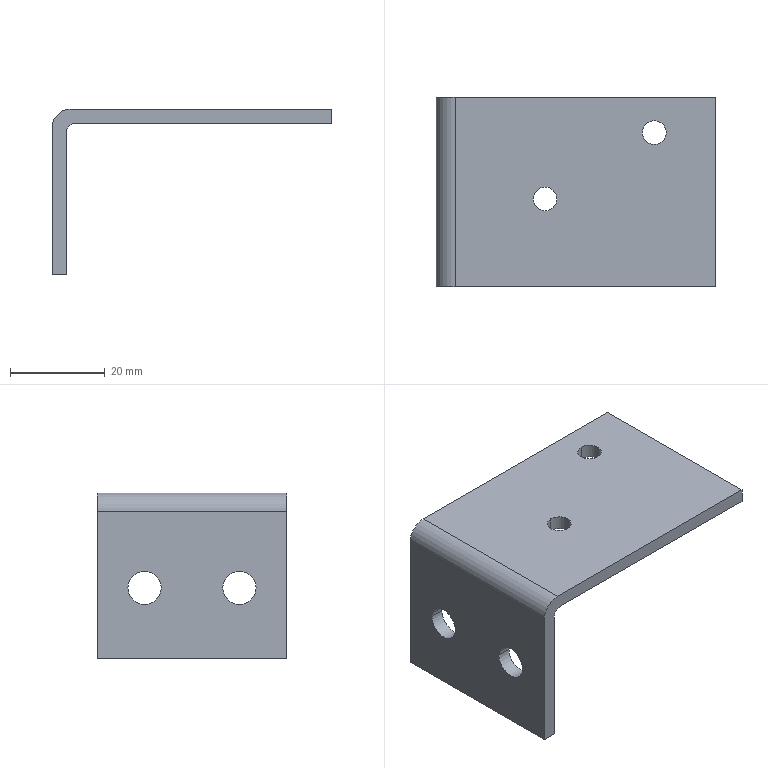Component | SolidWorks | 30-41A-1 | 1 solid | 18 faces | box 59 x 40 x 35 mm | volume 10468 mm3 | cylinder 10 | plane 8 | commonest cylinder face diameters 5 x4 7 x4 8 x1 4 x1
build123d program:
from build123d import *

# Parameters (mm, degrees)
EXTRUDE1_DEPTH        = 20
EXTRUDE1_DEPTH_BACK   = 20
SKETCH2_R             = 3.5
CUT_EXTRUDE1_DEPTH    = 20
M6_TAPPED_HOLE1_D     = 5
M6_TAPPED_HOLE1_DEPTH = 17
M6_TAPPED_HOLE1_TIP   = 1.502


with BuildPart() as part:
    # Sketch1 → Extrude1 (new, two sides: drawn at the far end of the back side and taken through both)
    with BuildSketch(Plane.XY.offset(-EXTRUDE1_DEPTH_BACK)):
        with BuildLine():
            Line((4, 0), (35, 0))
            Line((35, 0), (35, 3))
            Line((35, 3), (5, 3))
            ThreePointArc((5, 3), (3.586, 3.586), (3, 5))
            Line((3, 5), (3, 59))
            Line((3, 59), (0, 59))
            Line((0, 59), (0, 4))
            ThreePointArc((0, 4), (1.172, 1.172), (4, 0))
        make_face()
    extrude(amount=EXTRUDE1_DEPTH + EXTRUDE1_DEPTH_BACK)

    # Sketch2 → Cut-Extrude1 (cut)
    with BuildSketch(Plane(origin=(0, 3, 0), x_dir=(1, 0, 0), z_dir=(0, 1, 0))):
        with Locations(Location((20, 10, 0), (0, 0, 270))):
            Circle(SKETCH2_R)
        with Locations(Location((20, -10, 0), (0, 0, 90))):
            Circle(SKETCH2_R)
    extrude(amount=-CUT_EXTRUDE1_DEPTH, mode=Mode.SUBTRACT)

    # M6 Tapped Hole1
    with Locations(Plane.ZY):
        with Locations((-12.5, 46), (1.5, 23)):
            Hole(M6_TAPPED_HOLE1_D / 2, depth=M6_TAPPED_HOLE1_DEPTH)
            with Locations((0, 0, -(M6_TAPPED_HOLE1_DEPTH + M6_TAPPED_HOLE1_TIP / 2))):  # 118° drill point
                Cone(0, M6_TAPPED_HOLE1_D / 2, M6_TAPPED_HOLE1_TIP, mode=Mode.SUBTRACT)


solid = part.part

# Placed as in the assembly
solid = solid.moved(Location((-429.208, -117.092, 109.188), (90, 0, -90)))
STEP:
#1=CARTESIAN_POINT('',(-15.087,-4.216,4.181));
#2=VERTEX_POINT('',#1);
#3=CARTESIAN_POINT('',(-15.087,-4.019,4.181));
#4=VERTEX_POINT('',#3);
#5=CARTESIAN_POINT('',(-15.087,-4.118,4.181));
#6=DIRECTION('',(-0.,-0.,-1.));
#7=DIRECTION('',(1.,0.,0.));
#8=AXIS2_PLACEMENT_3D('',#5,#6,#7);
#9=CIRCLE('',#8,0.09843);
#10=EDGE_CURVE('',#2,#4,#9,.T.);
#11=ORIENTED_EDGE('',*,*,#10,.T.);
#12=CARTESIAN_POINT('',(-15.087,-4.019,4.299));
#13=VERTEX_POINT('',#12);
#14=CARTESIAN_POINT('',(-15.087,-4.019,4.299));
#15=DIRECTION('',(0.,0.,1.));
#16=VECTOR('',#15,39.37);
#17=LINE('',#14,#16);
#18=EDGE_CURVE('',#4,#13,#17,.T.);
#19=ORIENTED_EDGE('',*,*,#18,.T.);
#20=CARTESIAN_POINT('',(-15.087,-4.216,4.299));
#21=VERTEX_POINT('',#20);
#22=CARTESIAN_POINT('',(-15.087,-4.118,4.299));
#23=DIRECTION('',(0.,0.,1.));
#24=DIRECTION('',(0.,-1.,0.));
#25=AXIS2_PLACEMENT_3D('',#22,#23,#24);
#26=CIRCLE('',#25,0.09843);
#27=EDGE_CURVE('',#13,#21,#26,.T.);
#28=ORIENTED_EDGE('',*,*,#27,.T.);
#29=CARTESIAN_POINT('',(-15.087,-4.216,4.299));
#30=DIRECTION('',(0.,0.,1.));
#31=VECTOR('',#30,39.37);
#32=LINE('',#29,#31);
#33=EDGE_CURVE('',#2,#21,#32,.T.);
#34=ORIENTED_EDGE('',*,*,#33,.F.);
#35=EDGE_LOOP('',(#11,#19,#28,#34));
#36=FACE_OUTER_BOUND('',#35,.T.);
#37=CARTESIAN_POINT('',(-15.087,-4.118,4.299));
#38=DIRECTION('',(0.,0.,1.));
#39=DIRECTION('',(0.,-1.,0.));
#40=AXIS2_PLACEMENT_3D('',#37,#38,#39);
#41=CYLINDRICAL_SURFACE('',#40,0.09843);
#42=ADVANCED_FACE('',(#36),#41,.F.);
#43=CARTESIAN_POINT('',(-15.992,-4.767,4.181));
#44=VERTEX_POINT('',#43);
#45=CARTESIAN_POINT('',(-15.992,-4.571,4.181));
#46=VERTEX_POINT('',#45);
#47=CARTESIAN_POINT('',(-15.992,-4.669,4.181));
#48=DIRECTION('',(-0.,-0.,-1.));
#49=DIRECTION('',(1.,0.,0.));
#50=AXIS2_PLACEMENT_3D('',#47,#48,#49);
#51=CIRCLE('',#50,0.09843);
#52=EDGE_CURVE('',#44,#46,#51,.T.);
#53=ORIENTED_EDGE('',*,*,#52,.T.);
#54=CARTESIAN_POINT('',(-15.992,-4.571,4.299));
#55=VERTEX_POINT('',#54);
#56=CARTESIAN_POINT('',(-15.992,-4.571,4.299));
#57=DIRECTION('',(0.,0.,1.));
#58=VECTOR('',#57,39.37);
#59=LINE('',#56,#58);
#60=EDGE_CURVE('',#46,#55,#59,.T.);
#61=ORIENTED_EDGE('',*,*,#60,.T.);
#62=CARTESIAN_POINT('',(-15.992,-4.767,4.299));
#63=VERTEX_POINT('',#62);
#64=CARTESIAN_POINT('',(-15.992,-4.669,4.299));
#65=DIRECTION('',(0.,0.,1.));
#66=DIRECTION('',(0.,-1.,0.));
#67=AXIS2_PLACEMENT_3D('',#64,#65,#66);
#68=CIRCLE('',#67,0.09843);
#69=EDGE_CURVE('',#55,#63,#68,.T.);
#70=ORIENTED_EDGE('',*,*,#69,.T.);
#71=CARTESIAN_POINT('',(-15.992,-4.767,4.299));
#72=DIRECTION('',(0.,0.,1.));
#73=VECTOR('',#72,39.37);
#74=LINE('',#71,#73);
#75=EDGE_CURVE('',#44,#63,#74,.T.);
#76=ORIENTED_EDGE('',*,*,#75,.F.);
#77=EDGE_LOOP('',(#53,#61,#70,#76));
#78=FACE_OUTER_BOUND('',#77,.T.);
#79=CARTESIAN_POINT('',(-15.992,-4.669,4.299));
#80=DIRECTION('',(0.,0.,1.));
#81=DIRECTION('',(0.,-1.,0.));
#82=AXIS2_PLACEMENT_3D('',#79,#80,#81);
#83=CYLINDRICAL_SURFACE('',#82,0.09843);
#84=ADVANCED_FACE('',(#78),#83,.F.);
#85=CARTESIAN_POINT('',(-16.898,-5.141,3.511));
#86=VERTEX_POINT('',#85);
#87=CARTESIAN_POINT('',(-16.898,-4.866,3.511));
#88=VERTEX_POINT('',#87);
#89=CARTESIAN_POINT('',(-16.898,-5.004,3.511));
#90=DIRECTION('',(-1.,-0.,0.));
#91=DIRECTION('',(0.,1.,0.));
#92=AXIS2_PLACEMENT_3D('',#89,#90,#91);
#93=CIRCLE('',#92,0.1378);
#94=EDGE_CURVE('',#86,#88,#93,.T.);
#95=ORIENTED_EDGE('',*,*,#94,.T.);
#96=CARTESIAN_POINT('',(-16.78,-4.866,3.511));
#97=VERTEX_POINT('',#96);
#98=CARTESIAN_POINT('',(-17.567,-4.866,3.511));
#99=DIRECTION('',(1.,0.,-0.));
#100=VECTOR('',#99,39.37);
#101=LINE('',#98,#100);
#102=EDGE_CURVE('',#88,#97,#101,.T.);
#103=ORIENTED_EDGE('',*,*,#102,.T.);
#104=CARTESIAN_POINT('',(-16.78,-5.141,3.511));
#105=VERTEX_POINT('',#104);
#106=CARTESIAN_POINT('',(-16.78,-5.004,3.511));
#107=DIRECTION('',(1.,0.,-0.));
#108=DIRECTION('',(0.,1.,0.));
#109=AXIS2_PLACEMENT_3D('',#106,#107,#108);
#110=CIRCLE('',#109,0.1378);
#111=EDGE_CURVE('',#97,#105,#110,.T.);
#112=ORIENTED_EDGE('',*,*,#111,.T.);
#113=CARTESIAN_POINT('',(-17.567,-5.141,3.511));
#114=DIRECTION('',(1.,0.,-0.));
#115=VECTOR('',#114,39.37);
#116=LINE('',#113,#115);
#117=EDGE_CURVE('',#86,#105,#116,.T.);
#118=ORIENTED_EDGE('',*,*,#117,.F.);
#119=EDGE_LOOP('',(#95,#103,#112,#118));
#120=FACE_OUTER_BOUND('',#119,.T.);
#121=CARTESIAN_POINT('',(-17.567,-5.004,3.511));
#122=DIRECTION('',(1.,0.,-0.));
#123=DIRECTION('',(0.,-1.,0.));
#124=AXIS2_PLACEMENT_3D('',#121,#122,#123);
#125=CYLINDRICAL_SURFACE('',#124,0.1378);
#126=ADVANCED_FACE('',(#120),#125,.F.);
#127=CARTESIAN_POINT('',(-16.898,-4.354,3.511));
#128=VERTEX_POINT('',#127);
#129=CARTESIAN_POINT('',(-16.898,-4.078,3.511));
#130=VERTEX_POINT('',#129);
#131=CARTESIAN_POINT('',(-16.898,-4.216,3.511));
#132=DIRECTION('',(-1.,-0.,0.));
#133=DIRECTION('',(0.,1.,0.));
#134=AXIS2_PLACEMENT_3D('',#131,#132,#133);
#135=CIRCLE('',#134,0.1378);
#136=EDGE_CURVE('',#128,#130,#135,.T.);
#137=ORIENTED_EDGE('',*,*,#136,.T.);
#138=CARTESIAN_POINT('',(-16.78,-4.078,3.511));
#139=VERTEX_POINT('',#138);
#140=CARTESIAN_POINT('',(-17.567,-4.078,3.511));
#141=DIRECTION('',(1.,0.,-0.));
#142=VECTOR('',#141,39.37);
#143=LINE('',#140,#142);
#144=EDGE_CURVE('',#130,#139,#143,.T.);
#145=ORIENTED_EDGE('',*,*,#144,.T.);
#146=CARTESIAN_POINT('',(-16.78,-4.354,3.511));
#147=VERTEX_POINT('',#146);
#148=CARTESIAN_POINT('',(-16.78,-4.216,3.511));
#149=DIRECTION('',(1.,0.,-0.));
#150=DIRECTION('',(0.,-1.,0.));
#151=AXIS2_PLACEMENT_3D('',#148,#149,#150);
#152=CIRCLE('',#151,0.1378);
#153=EDGE_CURVE('',#139,#147,#152,.T.);
#154=ORIENTED_EDGE('',*,*,#153,.T.);
#155=CARTESIAN_POINT('',(-17.567,-4.354,3.511));
#156=DIRECTION('',(1.,0.,-0.));
#157=VECTOR('',#156,39.37);
#158=LINE('',#155,#157);
#159=EDGE_CURVE('',#128,#147,#158,.T.);
#160=ORIENTED_EDGE('',*,*,#159,.F.);
#161=EDGE_LOOP('',(#137,#145,#154,#160));
#162=FACE_OUTER_BOUND('',#161,.T.);
#163=CARTESIAN_POINT('',(-17.567,-4.216,3.511));
#164=DIRECTION('',(1.,0.,-0.));
#165=DIRECTION('',(0.,-1.,0.));
#166=AXIS2_PLACEMENT_3D('',#163,#164,#165);
#167=CYLINDRICAL_SURFACE('',#166,0.1378);
#168=ADVANCED_FACE('',(#162),#167,.F.);
#169=CARTESIAN_POINT('',(-16.78,-3.823,2.921));
#170=VERTEX_POINT('',#169);
#171=CARTESIAN_POINT('',(-16.78,-5.397,2.921));
#172=VERTEX_POINT('',#171);
#173=CARTESIAN_POINT('',(-16.78,-3.823,2.921));
#174=DIRECTION('',(0.,-1.,0.));
#175=VECTOR('',#174,39.37);
#176=LINE('',#173,#175);
#177=EDGE_CURVE('',#170,#172,#176,.T.);
#178=ORIENTED_EDGE('',*,*,#177,.T.);
#179=CARTESIAN_POINT('',(-16.898,-5.397,2.921));
#180=VERTEX_POINT('',#179);
#181=CARTESIAN_POINT('',(-16.898,-5.397,2.921));
#182=DIRECTION('',(1.,0.,-0.));
#183=VECTOR('',#182,39.37);
#184=LINE('',#181,#183);
#185=EDGE_CURVE('',#180,#172,#184,.T.);
#186=ORIENTED_EDGE('',*,*,#185,.F.);
#187=CARTESIAN_POINT('',(-16.898,-3.823,2.921));
#188=VERTEX_POINT('',#187);
#189=CARTESIAN_POINT('',(-16.898,-3.823,2.921));
#190=DIRECTION('',(0.,-1.,0.));
#191=VECTOR('',#190,39.37);
#192=LINE('',#189,#191);
#193=EDGE_CURVE('',#188,#180,#192,.T.);
#194=ORIENTED_EDGE('',*,*,#193,.F.);
#195=CARTESIAN_POINT('',(-16.898,-3.823,2.921));
#196=DIRECTION('',(1.,0.,-0.));
#197=VECTOR('',#196,39.37);
#198=LINE('',#195,#197);
#199=EDGE_CURVE('',#188,#170,#198,.T.);
#200=ORIENTED_EDGE('',*,*,#199,.T.);
#201=EDGE_LOOP('',(#178,#186,#194,#200));
#202=FACE_OUTER_BOUND('',#201,.T.);
#203=CARTESIAN_POINT('',(-16.898,-3.823,2.921));
#204=DIRECTION('',(-0.,-0.,-1.));
#205=DIRECTION('',(-0.,1.,-0.));
#206=AXIS2_PLACEMENT_3D('',#203,#204,#205);
#207=PLANE('',#206);
#208=ADVANCED_FACE('',(#202),#207,.T.);
#209=ORIENTED_EDGE('',*,*,#94,.F.);
#210=CARTESIAN_POINT('',(-16.898,-5.004,3.511));
#211=DIRECTION('',(-1.,-0.,0.));
#212=DIRECTION('',(0.,1.,0.));
#213=AXIS2_PLACEMENT_3D('',#210,#211,#212);
#214=CIRCLE('',#213,0.1378);
#215=EDGE_CURVE('',#88,#86,#214,.T.);
#216=ORIENTED_EDGE('',*,*,#215,.F.);
#217=EDGE_LOOP('',(#209,#216));
#218=FACE_BOUND('',#217,.T.);
#219=ORIENTED_EDGE('',*,*,#136,.F.);
#220=CARTESIAN_POINT('',(-16.898,-4.216,3.511));
#221=DIRECTION('',(-1.,-0.,0.));
#222=DIRECTION('',(0.,1.,0.));
#223=AXIS2_PLACEMENT_3D('',#220,#221,#222);
#224=CIRCLE('',#223,0.1378);
#225=EDGE_CURVE('',#130,#128,#224,.T.);
#226=ORIENTED_EDGE('',*,*,#225,.F.);
#227=EDGE_LOOP('',(#219,#226));
#228=FACE_BOUND('',#227,.T.);
#229=ORIENTED_EDGE('',*,*,#193,.T.);
#230=CARTESIAN_POINT('',(-16.898,-5.397,4.141));
#231=VERTEX_POINT('',#230);
#232=CARTESIAN_POINT('',(-16.898,-5.397,4.141));
#233=DIRECTION('',(-0.,-0.,-1.));
#234=VECTOR('',#233,39.37);
#235=LINE('',#232,#234);
#236=EDGE_CURVE('',#231,#180,#235,.T.);
#237=ORIENTED_EDGE('',*,*,#236,.F.);
#238=CARTESIAN_POINT('',(-16.898,-3.823,4.141));
#239=VERTEX_POINT('',#238);
#240=CARTESIAN_POINT('',(-16.898,-3.823,4.141));
#241=DIRECTION('',(0.,-1.,0.));
#242=VECTOR('',#241,39.37);
#243=LINE('',#240,#242);
#244=EDGE_CURVE('',#239,#231,#243,.T.);
#245=ORIENTED_EDGE('',*,*,#244,.F.);
#246=CARTESIAN_POINT('',(-16.898,-3.823,4.141));
#247=DIRECTION('',(-0.,-0.,-1.));
#248=VECTOR('',#247,39.37);
#249=LINE('',#246,#248);
#250=EDGE_CURVE('',#239,#188,#249,.T.);
#251=ORIENTED_EDGE('',*,*,#250,.T.);
#252=EDGE_LOOP('',(#229,#237,#245,#251));
#253=FACE_OUTER_BOUND('',#252,.T.);
#254=CARTESIAN_POINT('',(-16.898,-3.823,4.141));
#255=DIRECTION('',(-1.,-0.,0.));
#256=DIRECTION('',(-0.,1.,-0.));
#257=AXIS2_PLACEMENT_3D('',#254,#255,#256);
#258=PLANE('',#257);
#259=ADVANCED_FACE('',(#218,#228,#253),#258,.T.);
#260=ORIENTED_EDGE('',*,*,#244,.T.);
#261=CARTESIAN_POINT('',(-16.74,-5.397,4.299));
#262=VERTEX_POINT('',#261);
#263=CARTESIAN_POINT('',(-16.74,-5.397,4.141));
#264=DIRECTION('',(0.,-1.,0.));
#265=DIRECTION('',(0.,0.,1.));
#266=AXIS2_PLACEMENT_3D('',#263,#264,#265);
#267=CIRCLE('',#266,0.1575);
#268=EDGE_CURVE('',#262,#231,#267,.T.);
#269=ORIENTED_EDGE('',*,*,#268,.F.);
#270=CARTESIAN_POINT('',(-16.74,-3.823,4.299));
#271=VERTEX_POINT('',#270);
#272=CARTESIAN_POINT('',(-16.74,-3.823,4.299));
#273=DIRECTION('',(0.,-1.,0.));
#274=VECTOR('',#273,39.37);
#275=LINE('',#272,#274);
#276=EDGE_CURVE('',#271,#262,#275,.T.);
#277=ORIENTED_EDGE('',*,*,#276,.F.);
#278=CARTESIAN_POINT('',(-16.74,-3.823,4.141));
#279=DIRECTION('',(0.,-1.,0.));
#280=DIRECTION('',(0.,0.,1.));
#281=AXIS2_PLACEMENT_3D('',#278,#279,#280);
#282=CIRCLE('',#281,0.1575);
#283=EDGE_CURVE('',#271,#239,#282,.T.);
#284=ORIENTED_EDGE('',*,*,#283,.T.);
#285=EDGE_LOOP('',(#260,#269,#277,#284));
#286=FACE_OUTER_BOUND('',#285,.T.);
#287=CARTESIAN_POINT('',(-16.74,-3.823,4.141));
#288=DIRECTION('',(0.,-1.,0.));
#289=DIRECTION('',(0.,0.,-1.));
#290=AXIS2_PLACEMENT_3D('',#287,#288,#289);
#291=CYLINDRICAL_SURFACE('',#290,0.1575);
#292=ADVANCED_FACE('',(#286),#291,.T.);
#293=CARTESIAN_POINT('',(-15.087,-4.118,4.299));
#294=DIRECTION('',(0.,0.,1.));
#295=DIRECTION('',(0.,-1.,0.));
#296=AXIS2_PLACEMENT_3D('',#293,#294,#295);
#297=CIRCLE('',#296,0.09843);
#298=EDGE_CURVE('',#21,#13,#297,.T.);
#299=ORIENTED_EDGE('',*,*,#298,.F.);
#300=ORIENTED_EDGE('',*,*,#27,.F.);
#301=EDGE_LOOP('',(#299,#300));
#302=FACE_BOUND('',#301,.T.);
#303=CARTESIAN_POINT('',(-15.992,-4.669,4.299));
#304=DIRECTION('',(0.,0.,1.));
#305=DIRECTION('',(0.,-1.,0.));
#306=AXIS2_PLACEMENT_3D('',#303,#304,#305);
#307=CIRCLE('',#306,0.09843);
#308=EDGE_CURVE('',#63,#55,#307,.T.);
#309=ORIENTED_EDGE('',*,*,#308,.F.);
#310=ORIENTED_EDGE('',*,*,#69,.F.);
#311=EDGE_LOOP('',(#309,#310));
#312=FACE_BOUND('',#311,.T.);
#313=ORIENTED_EDGE('',*,*,#276,.T.);
#314=CARTESIAN_POINT('',(-14.575,-5.397,4.299));
#315=VERTEX_POINT('',#314);
#316=CARTESIAN_POINT('',(-16.74,-5.397,4.299));
#317=DIRECTION('',(-1.,-0.,0.));
#318=VECTOR('',#317,39.37);
#319=LINE('',#316,#318);
#320=EDGE_CURVE('',#315,#262,#319,.T.);
#321=ORIENTED_EDGE('',*,*,#320,.F.);
#322=CARTESIAN_POINT('',(-14.575,-3.823,4.299));
#323=VERTEX_POINT('',#322);
#324=CARTESIAN_POINT('',(-14.575,-3.823,4.299));
#325=DIRECTION('',(0.,-1.,0.));
#326=VECTOR('',#325,39.37);
#327=LINE('',#324,#326);
#328=EDGE_CURVE('',#323,#315,#327,.T.);
#329=ORIENTED_EDGE('',*,*,#328,.F.);
#330=CARTESIAN_POINT('',(-16.74,-3.823,4.299));
#331=DIRECTION('',(-1.,-0.,0.));
#332=VECTOR('',#331,39.37);
#333=LINE('',#330,#332);
#334=EDGE_CURVE('',#323,#271,#333,.T.);
#335=ORIENTED_EDGE('',*,*,#334,.T.);
#336=EDGE_LOOP('',(#313,#321,#329,#335));
#337=FACE_OUTER_BOUND('',#336,.T.);
#338=CARTESIAN_POINT('',(-16.74,-3.823,4.299));
#339=DIRECTION('',(0.,0.,1.));
#340=DIRECTION('',(0.,-1.,0.));
#341=AXIS2_PLACEMENT_3D('',#338,#339,#340);
#342=PLANE('',#341);
#343=ADVANCED_FACE('',(#302,#312,#337),#342,.T.);
#344=ORIENTED_EDGE('',*,*,#328,.T.);
#345=CARTESIAN_POINT('',(-14.575,-5.397,4.181));
#346=VERTEX_POINT('',#345);
#347=CARTESIAN_POINT('',(-14.575,-5.397,4.299));
#348=DIRECTION('',(0.,0.,1.));
#349=VECTOR('',#348,39.37);
#350=LINE('',#347,#349);
#351=EDGE_CURVE('',#346,#315,#350,.T.);
#352=ORIENTED_EDGE('',*,*,#351,.F.);
#353=CARTESIAN_POINT('',(-14.575,-3.823,4.181));
#354=VERTEX_POINT('',#353);
#355=CARTESIAN_POINT('',(-14.575,-3.823,4.181));
#356=DIRECTION('',(0.,-1.,0.));
#357=VECTOR('',#356,39.37);
#358=LINE('',#355,#357);
#359=EDGE_CURVE('',#354,#346,#358,.T.);
#360=ORIENTED_EDGE('',*,*,#359,.F.);
#361=CARTESIAN_POINT('',(-14.575,-3.823,4.299));
#362=DIRECTION('',(0.,0.,1.));
#363=VECTOR('',#362,39.37);
#364=LINE('',#361,#363);
#365=EDGE_CURVE('',#354,#323,#364,.T.);
#366=ORIENTED_EDGE('',*,*,#365,.T.);
#367=EDGE_LOOP('',(#344,#352,#360,#366));
#368=FACE_OUTER_BOUND('',#367,.T.);
#369=CARTESIAN_POINT('',(-14.575,-3.823,4.299));
#370=DIRECTION('',(1.,0.,-0.));
#371=DIRECTION('',(0.,-1.,0.));
#372=AXIS2_PLACEMENT_3D('',#369,#370,#371);
#373=PLANE('',#372);
#374=ADVANCED_FACE('',(#368),#373,.T.);
#375=ORIENTED_EDGE('',*,*,#10,.F.);
#376=CARTESIAN_POINT('',(-15.087,-4.118,4.181));
#377=DIRECTION('',(-0.,-0.,-1.));
#378=DIRECTION('',(1.,0.,0.));
#379=AXIS2_PLACEMENT_3D('',#376,#377,#378);
#380=CIRCLE('',#379,0.09843);
#381=EDGE_CURVE('',#4,#2,#380,.T.);
#382=ORIENTED_EDGE('',*,*,#381,.F.);
#383=EDGE_LOOP('',(#375,#382));
#384=FACE_BOUND('',#383,.T.);
#385=ORIENTED_EDGE('',*,*,#52,.F.);
#386=CARTESIAN_POINT('',(-15.992,-4.669,4.181));
#387=DIRECTION('',(-0.,-0.,-1.));
#388=DIRECTION('',(1.,0.,0.));
#389=AXIS2_PLACEMENT_3D('',#386,#387,#388);
#390=CIRCLE('',#389,0.09843);
#391=EDGE_CURVE('',#46,#44,#390,.T.);
#392=ORIENTED_EDGE('',*,*,#391,.F.);
#393=EDGE_LOOP('',(#385,#392));
#394=FACE_BOUND('',#393,.T.);
#395=ORIENTED_EDGE('',*,*,#359,.T.);
#396=CARTESIAN_POINT('',(-16.701,-5.397,4.181));
#397=VERTEX_POINT('',#396);
#398=CARTESIAN_POINT('',(-14.575,-5.397,4.181));
#399=DIRECTION('',(1.,0.,-0.));
#400=VECTOR('',#399,39.37);
#401=LINE('',#398,#400);
#402=EDGE_CURVE('',#397,#346,#401,.T.);
#403=ORIENTED_EDGE('',*,*,#402,.F.);
#404=CARTESIAN_POINT('',(-16.701,-3.823,4.181));
#405=VERTEX_POINT('',#404);
#406=CARTESIAN_POINT('',(-16.701,-3.823,4.181));
#407=DIRECTION('',(0.,-1.,0.));
#408=VECTOR('',#407,39.37);
#409=LINE('',#406,#408);
#410=EDGE_CURVE('',#405,#397,#409,.T.);
#411=ORIENTED_EDGE('',*,*,#410,.F.);
#412=CARTESIAN_POINT('',(-14.575,-3.823,4.181));
#413=DIRECTION('',(1.,0.,-0.));
#414=VECTOR('',#413,39.37);
#415=LINE('',#412,#414);
#416=EDGE_CURVE('',#405,#354,#415,.T.);
#417=ORIENTED_EDGE('',*,*,#416,.T.);
#418=EDGE_LOOP('',(#395,#403,#411,#417));
#419=FACE_OUTER_BOUND('',#418,.T.);
#420=CARTESIAN_POINT('',(-14.575,-3.823,4.181));
#421=DIRECTION('',(-0.,-0.,-1.));
#422=DIRECTION('',(1.,0.,-0.));
#423=AXIS2_PLACEMENT_3D('',#420,#421,#422);
#424=PLANE('',#423);
#425=ADVANCED_FACE('',(#384,#394,#419),#424,.T.);
#426=ORIENTED_EDGE('',*,*,#410,.T.);
#427=CARTESIAN_POINT('',(-16.78,-5.397,4.102));
#428=VERTEX_POINT('',#427);
#429=CARTESIAN_POINT('',(-16.701,-5.397,4.102));
#430=DIRECTION('',(-0.,1.,-0.));
#431=DIRECTION('',(0.,0.,1.));
#432=AXIS2_PLACEMENT_3D('',#429,#430,#431);
#433=CIRCLE('',#432,0.07874);
#434=EDGE_CURVE('',#428,#397,#433,.T.);
#435=ORIENTED_EDGE('',*,*,#434,.F.);
#436=CARTESIAN_POINT('',(-16.78,-3.823,4.102));
#437=VERTEX_POINT('',#436);
#438=CARTESIAN_POINT('',(-16.78,-3.823,4.102));
#439=DIRECTION('',(0.,-1.,0.));
#440=VECTOR('',#439,39.37);
#441=LINE('',#438,#440);
#442=EDGE_CURVE('',#437,#428,#441,.T.);
#443=ORIENTED_EDGE('',*,*,#442,.F.);
#444=CARTESIAN_POINT('',(-16.701,-3.823,4.102));
#445=DIRECTION('',(-0.,1.,-0.));
#446=DIRECTION('',(0.,0.,1.));
#447=AXIS2_PLACEMENT_3D('',#444,#445,#446);
#448=CIRCLE('',#447,0.07874);
#449=EDGE_CURVE('',#437,#405,#448,.T.);
#450=ORIENTED_EDGE('',*,*,#449,.T.);
#451=EDGE_LOOP('',(#426,#435,#443,#450));
#452=FACE_OUTER_BOUND('',#451,.T.);
#453=CARTESIAN_POINT('',(-16.701,-3.823,4.102));
#454=DIRECTION('',(0.,-1.,0.));
#455=DIRECTION('',(0.,0.,-1.));
#456=AXIS2_PLACEMENT_3D('',#453,#454,#455);
#457=CYLINDRICAL_SURFACE('',#456,0.07874);
#458=ADVANCED_FACE('',(#452),#457,.F.);
#459=CARTESIAN_POINT('',(-16.78,-5.004,3.511));
#460=DIRECTION('',(1.,0.,-0.));
#461=DIRECTION('',(0.,1.,0.));
#462=AXIS2_PLACEMENT_3D('',#459,#460,#461);
#463=CIRCLE('',#462,0.1378);
#464=EDGE_CURVE('',#105,#97,#463,.T.);
#465=ORIENTED_EDGE('',*,*,#464,.F.);
#466=ORIENTED_EDGE('',*,*,#111,.F.);
#467=EDGE_LOOP('',(#465,#466));
#468=FACE_BOUND('',#467,.T.);
#469=CARTESIAN_POINT('',(-16.78,-4.216,3.511));
#470=DIRECTION('',(1.,0.,-0.));
#471=DIRECTION('',(0.,-1.,0.));
#472=AXIS2_PLACEMENT_3D('',#469,#470,#471);
#473=CIRCLE('',#472,0.1378);
#474=EDGE_CURVE('',#147,#139,#473,.T.);
#475=ORIENTED_EDGE('',*,*,#474,.F.);
#476=ORIENTED_EDGE('',*,*,#153,.F.);
#477=EDGE_LOOP('',(#475,#476));
#478=FACE_BOUND('',#477,.T.);
#479=ORIENTED_EDGE('',*,*,#442,.T.);
#480=CARTESIAN_POINT('',(-16.78,-5.397,4.102));
#481=DIRECTION('',(0.,0.,1.));
#482=VECTOR('',#481,39.37);
#483=LINE('',#480,#482);
#484=EDGE_CURVE('',#172,#428,#483,.T.);
#485=ORIENTED_EDGE('',*,*,#484,.F.);
#486=ORIENTED_EDGE('',*,*,#177,.F.);
#487=CARTESIAN_POINT('',(-16.78,-3.823,4.102));
#488=DIRECTION('',(0.,0.,1.));
#489=VECTOR('',#488,39.37);
#490=LINE('',#487,#489);
#491=EDGE_CURVE('',#170,#437,#490,.T.);
#492=ORIENTED_EDGE('',*,*,#491,.T.);
#493=EDGE_LOOP('',(#479,#485,#486,#492));
#494=FACE_OUTER_BOUND('',#493,.T.);
#495=CARTESIAN_POINT('',(-16.78,-3.823,4.102));
#496=DIRECTION('',(1.,0.,-0.));
#497=DIRECTION('',(0.,-1.,0.));
#498=AXIS2_PLACEMENT_3D('',#495,#496,#497);
#499=PLANE('',#498);
#500=ADVANCED_FACE('',(#468,#478,#494),#499,.T.);
#501=ORIENTED_EDGE('',*,*,#199,.F.);
#502=ORIENTED_EDGE('',*,*,#250,.F.);
#503=ORIENTED_EDGE('',*,*,#283,.F.);
#504=ORIENTED_EDGE('',*,*,#334,.F.);
#505=ORIENTED_EDGE('',*,*,#365,.F.);
#506=ORIENTED_EDGE('',*,*,#416,.F.);
#507=ORIENTED_EDGE('',*,*,#449,.F.);
#508=ORIENTED_EDGE('',*,*,#491,.F.);
#509=EDGE_LOOP('',(#501,#502,#503,#504,#505,#506,#507,#508));
#510=FACE_OUTER_BOUND('',#509,.T.);
#511=CARTESIAN_POINT('',(-16.701,-3.823,4.102));
#512=DIRECTION('',(-0.,1.,-0.));
#513=DIRECTION('',(0.,0.,1.));
#514=AXIS2_PLACEMENT_3D('',#511,#512,#513);
#515=PLANE('',#514);
#516=ADVANCED_FACE('',(#510),#515,.T.);
#517=ORIENTED_EDGE('',*,*,#185,.T.);
#518=ORIENTED_EDGE('',*,*,#484,.T.);
#519=ORIENTED_EDGE('',*,*,#434,.T.);
#520=ORIENTED_EDGE('',*,*,#402,.T.);
#521=ORIENTED_EDGE('',*,*,#351,.T.);
#522=ORIENTED_EDGE('',*,*,#320,.T.);
#523=ORIENTED_EDGE('',*,*,#268,.T.);
#524=ORIENTED_EDGE('',*,*,#236,.T.);
#525=EDGE_LOOP('',(#517,#518,#519,#520,#521,#522,#523,#524));
#526=FACE_OUTER_BOUND('',#525,.T.);
#527=CARTESIAN_POINT('',(-16.701,-5.397,4.102));
#528=DIRECTION('',(-0.,1.,-0.));
#529=DIRECTION('',(0.,0.,1.));
#530=AXIS2_PLACEMENT_3D('',#527,#528,#529);
#531=PLANE('',#530);
#532=ADVANCED_FACE('',(#526),#531,.F.);
#533=ORIENTED_EDGE('',*,*,#144,.F.);
#534=ORIENTED_EDGE('',*,*,#225,.T.);
#535=ORIENTED_EDGE('',*,*,#159,.T.);
#536=ORIENTED_EDGE('',*,*,#474,.T.);
#537=EDGE_LOOP('',(#533,#534,#535,#536));
#538=FACE_OUTER_BOUND('',#537,.T.);
#539=CARTESIAN_POINT('',(-17.567,-4.216,3.511));
#540=DIRECTION('',(1.,0.,-0.));
#541=DIRECTION('',(0.,-1.,0.));
#542=AXIS2_PLACEMENT_3D('',#539,#540,#541);
#543=CYLINDRICAL_SURFACE('',#542,0.1378);
#544=ADVANCED_FACE('',(#538),#543,.F.);
#545=ORIENTED_EDGE('',*,*,#102,.F.);
#546=ORIENTED_EDGE('',*,*,#215,.T.);
#547=ORIENTED_EDGE('',*,*,#117,.T.);
#548=ORIENTED_EDGE('',*,*,#464,.T.);
#549=EDGE_LOOP('',(#545,#546,#547,#548));
#550=FACE_OUTER_BOUND('',#549,.T.);
#551=CARTESIAN_POINT('',(-17.567,-5.004,3.511));
#552=DIRECTION('',(1.,0.,-0.));
#553=DIRECTION('',(0.,-1.,0.));
#554=AXIS2_PLACEMENT_3D('',#551,#552,#553);
#555=CYLINDRICAL_SURFACE('',#554,0.1378);
#556=ADVANCED_FACE('',(#550),#555,.F.);
#557=ORIENTED_EDGE('',*,*,#60,.F.);
#558=ORIENTED_EDGE('',*,*,#391,.T.);
#559=ORIENTED_EDGE('',*,*,#75,.T.);
#560=ORIENTED_EDGE('',*,*,#308,.T.);
#561=EDGE_LOOP('',(#557,#558,#559,#560));
#562=FACE_OUTER_BOUND('',#561,.T.);
#563=CARTESIAN_POINT('',(-15.992,-4.669,4.299));
#564=DIRECTION('',(0.,0.,1.));
#565=DIRECTION('',(0.,-1.,0.));
#566=AXIS2_PLACEMENT_3D('',#563,#564,#565);
#567=CYLINDRICAL_SURFACE('',#566,0.09843);
#568=ADVANCED_FACE('',(#562),#567,.F.);
#569=ORIENTED_EDGE('',*,*,#18,.F.);
#570=ORIENTED_EDGE('',*,*,#381,.T.);
#571=ORIENTED_EDGE('',*,*,#33,.T.);
#572=ORIENTED_EDGE('',*,*,#298,.T.);
#573=EDGE_LOOP('',(#569,#570,#571,#572));
#574=FACE_OUTER_BOUND('',#573,.T.);
#575=CARTESIAN_POINT('',(-15.087,-4.118,4.299));
#576=DIRECTION('',(0.,0.,1.));
#577=DIRECTION('',(0.,-1.,0.));
#578=AXIS2_PLACEMENT_3D('',#575,#576,#577);
#579=CYLINDRICAL_SURFACE('',#578,0.09843);
#580=ADVANCED_FACE('',(#574),#579,.F.);
#581=CLOSED_SHELL('',(#42,#84,#126,#168,#208,#259,#292,#343,#374,#425,#458,#500,#516,#532,#544,#556,#568,#580));
#582=MANIFOLD_SOLID_BREP('',#581);
#583=CARTESIAN_POINT('',(0.,0.,0.));
#584=DIRECTION('',(0.,0.,1.));
#585=DIRECTION('',(1.,0.,0.));
#586=AXIS2_PLACEMENT_3D('',#583,#584,#585);
#587=(LENGTH_UNIT()NAMED_UNIT(*)SI_UNIT($,.METRE.));
#588=LENGTH_MEASURE_WITH_UNIT(LENGTH_MEASURE(0.0254),#587);
#589=DIMENSIONAL_EXPONENTS(1.,0.,0.,0.,0.,0.,0.);
#590=(CONVERSION_BASED_UNIT('',#588)LENGTH_UNIT()NAMED_UNIT(#589));
#591=UNCERTAINTY_MEASURE_WITH_UNIT(LENGTH_MEASURE(0.00001),#590,'','');
#592=(NAMED_UNIT(*)PLANE_ANGLE_UNIT()SI_UNIT($,.RADIAN.));
#593=(NAMED_UNIT(*)SI_UNIT($,.STERADIAN.)SOLID_ANGLE_UNIT());
#594=(GEOMETRIC_REPRESENTATION_CONTEXT(3)GLOBAL_UNCERTAINTY_ASSIGNED_CONTEXT((#591))GLOBAL_UNIT_ASSIGNED_CONTEXT((#590,#592,#593))REPRESENTATION_CONTEXT('',''));
#595=ADVANCED_BREP_SHAPE_REPRESENTATION('',(#582,#586),#594);
#596=COLOUR_RGB('',0.7922,0.8196,0.9333);
#597=FILL_AREA_STYLE_COLOUR('',#596);
#598=FILL_AREA_STYLE('',(#597));
#599=SURFACE_STYLE_FILL_AREA(#598);
#600=SURFACE_SIDE_STYLE('',(#599));
#601=SURFACE_STYLE_USAGE(.BOTH.,#600);
#602=PRESENTATION_STYLE_ASSIGNMENT((#601));
#603=STYLED_ITEM('',(#602),#582);
#604=PRESENTATION_LAYER_ASSIGNMENT('','',(#603));
#605=(LENGTH_UNIT()NAMED_UNIT(*)SI_UNIT($,.METRE.));
#606=LENGTH_MEASURE_WITH_UNIT(LENGTH_MEASURE(0.0254),#605);
#607=DIMENSIONAL_EXPONENTS(1.,0.,0.,0.,0.,0.,0.);
#608=(CONVERSION_BASED_UNIT('',#606)LENGTH_UNIT()NAMED_UNIT(#607));
#609=UNCERTAINTY_MEASURE_WITH_UNIT(LENGTH_MEASURE(0.00001),#608,'','');
#610=(NAMED_UNIT(*)PLANE_ANGLE_UNIT()SI_UNIT($,.RADIAN.));
#611=(NAMED_UNIT(*)SI_UNIT($,.STERADIAN.)SOLID_ANGLE_UNIT());
#612=(GEOMETRIC_REPRESENTATION_CONTEXT(3)GLOBAL_UNCERTAINTY_ASSIGNED_CONTEXT((#609))GLOBAL_UNIT_ASSIGNED_CONTEXT((#608,#610,#611))REPRESENTATION_CONTEXT('',''));
#613=MECHANICAL_DESIGN_GEOMETRIC_PRESENTATION_REPRESENTATION('',(#603),#612);